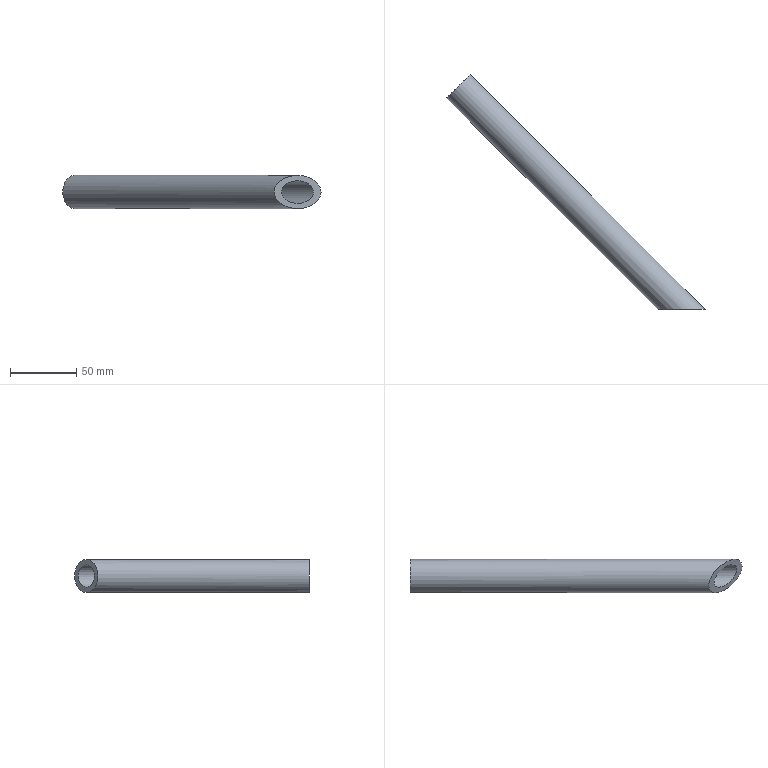Component | NX | BASE_FRAME_RND_TUBE_2 | 1 solid | 4 faces | box 194.45 x 176.78 x 25 mm | volume 62675 mm3 | plane 2 | cylinder 2 | commonest cylinder face diameters 25 x1 17 x1
STEP:
#1=CARTESIAN_POINT('',(0.,0.,0.));
#2=DIRECTION('',(0.,0.,1.));
#3=DIRECTION('',(1.,0.,0.));
#4=AXIS2_PLACEMENT_3D('',#1,#2,#3);
#5=CARTESIAN_POINT('',(-164.616,217.938,-371.5));
#6=VERTEX_POINT('',#5);
#7=CARTESIAN_POINT('',(-164.616,217.938,-380.));
#8=DIRECTION('',(0.7071,-0.7071,0.));
#9=DIRECTION('',(0.,0.,1.));
#10=AXIS2_PLACEMENT_3D('',#7,#8,#9);
#11=CIRCLE('',#10,8.5);
#12=CARTESIAN_POINT('',(-164.616,217.938,-380.));
#13=DIRECTION('',(-0.7071,0.7071,0.));
#14=DIRECTION('',(0.,0.,1.));
#15=AXIS2_PLACEMENT_3D('',#12,#13,#14);
#16=PLANE('',#15);
#17=CARTESIAN_POINT('',(8.5,0.));
#18=CARTESIAN_POINT('',(8.5,-14.722));
#19=CARTESIAN_POINT('',(-4.25,-7.361));
#20=CARTESIAN_POINT('',(-17.,-0.));
#21=CARTESIAN_POINT('',(-4.25,7.361));
#22=CARTESIAN_POINT('',(8.5,14.722));
#23=CARTESIAN_POINT('',(8.5,0.));
#24=(BOUNDED_CURVE()B_SPLINE_CURVE(2,(#17,#18,#19,#20,#21,#22,#23),.UNSPECIFIED.,.T.,.F.)B_SPLINE_CURVE_WITH_KNOTS((1,2,2,2,2,1),(-2.094,0.,2.094,4.189,6.283,8.378),.UNSPECIFIED.)CURVE()GEOMETRIC_REPRESENTATION_ITEM()RATIONAL_B_SPLINE_CURVE((1.,0.5,1.,0.5,1.,0.5,1.))REPRESENTATION_ITEM(''));
#25=(GEOMETRIC_REPRESENTATION_CONTEXT(2)PARAMETRIC_REPRESENTATION_CONTEXT()REPRESENTATION_CONTEXT('',''));
#26=DEFINITIONAL_REPRESENTATION('',(#24),#25);
#27=PCURVE('',#16,#26);
#28=CARTESIAN_POINT('',(12.161,41.161,-380.));
#29=DIRECTION('',(-0.7071,0.7071,0.));
#30=DIRECTION('',(0.,0.,1.));
#31=AXIS2_PLACEMENT_3D('',#28,#29,#30);
#32=CYLINDRICAL_SURFACE('',#31,8.5);
#33=CARTESIAN_POINT('',(6.283,250.));
#34=DIRECTION('',(-1.,0.));
#35=VECTOR('',#34,1.);
#36=LINE('',#33,#35);
#37=(GEOMETRIC_REPRESENTATION_CONTEXT(2)PARAMETRIC_REPRESENTATION_CONTEXT()REPRESENTATION_CONTEXT('',''));
#38=DEFINITIONAL_REPRESENTATION('',(#36),#37);
#39=PCURVE('',#32,#38);
#40=SURFACE_CURVE('',#11,(#27,#39),.PCURVE_S1.);
#41=EDGE_CURVE('',#6,#6,#40,.T.);
#42=ORIENTED_EDGE('',*,*,#41,.T.);
#43=EDGE_LOOP('',(#42));
#44=FACE_BOUND('',#43,.T.);
#45=CARTESIAN_POINT('',(-164.616,217.938,-367.5));
#46=VERTEX_POINT('',#45);
#47=CARTESIAN_POINT('',(-164.616,217.938,-380.));
#48=DIRECTION('',(0.7071,-0.7071,0.));
#49=DIRECTION('',(0.,0.,1.));
#50=AXIS2_PLACEMENT_3D('',#47,#48,#49);
#51=CIRCLE('',#50,12.5);
#52=CARTESIAN_POINT('',(12.5,0.));
#53=CARTESIAN_POINT('',(12.5,-21.651));
#54=CARTESIAN_POINT('',(-6.25,-10.825));
#55=CARTESIAN_POINT('',(-25.,-0.));
#56=CARTESIAN_POINT('',(-6.25,10.825));
#57=CARTESIAN_POINT('',(12.5,21.651));
#58=CARTESIAN_POINT('',(12.5,0.));
#59=(BOUNDED_CURVE()B_SPLINE_CURVE(2,(#52,#53,#54,#55,#56,#57,#58),.UNSPECIFIED.,.T.,.F.)B_SPLINE_CURVE_WITH_KNOTS((1,2,2,2,2,1),(-2.094,0.,2.094,4.189,6.283,8.378),.UNSPECIFIED.)CURVE()GEOMETRIC_REPRESENTATION_ITEM()RATIONAL_B_SPLINE_CURVE((1.,0.5,1.,0.5,1.,0.5,1.))REPRESENTATION_ITEM(''));
#60=(GEOMETRIC_REPRESENTATION_CONTEXT(2)PARAMETRIC_REPRESENTATION_CONTEXT()REPRESENTATION_CONTEXT('',''));
#61=DEFINITIONAL_REPRESENTATION('',(#59),#60);
#62=PCURVE('',#16,#61);
#63=CARTESIAN_POINT('',(12.161,41.161,-380.));
#64=DIRECTION('',(-0.7071,0.7071,0.));
#65=DIRECTION('',(0.,0.,1.));
#66=AXIS2_PLACEMENT_3D('',#63,#64,#65);
#67=CYLINDRICAL_SURFACE('',#66,12.5);
#68=CARTESIAN_POINT('',(6.283,250.));
#69=DIRECTION('',(-1.,0.));
#70=VECTOR('',#69,1.);
#71=LINE('',#68,#70);
#72=(GEOMETRIC_REPRESENTATION_CONTEXT(2)PARAMETRIC_REPRESENTATION_CONTEXT()REPRESENTATION_CONTEXT('',''));
#73=DEFINITIONAL_REPRESENTATION('',(#71),#72);
#74=PCURVE('',#67,#73);
#75=SURFACE_CURVE('',#51,(#62,#74),.PCURVE_S1.);
#76=EDGE_CURVE('',#46,#46,#75,.T.);
#77=ORIENTED_EDGE('',*,*,#76,.F.);
#78=EDGE_LOOP('',(#77));
#79=FACE_BOUND('',#78,.T.);
#80=ADVANCED_FACE('',(#44,#79),#16,.T.);
#81=CARTESIAN_POINT('',(3.322,50.,-367.5));
#82=VERTEX_POINT('',#81);
#83=CARTESIAN_POINT('',(-14.355,50.,-380.));
#84=VERTEX_POINT('',#83);
#85=CARTESIAN_POINT('',(3.322,50.,-380.));
#86=DIRECTION('',(0.,-1.,0.));
#87=DIRECTION('',(-1.,-0.,0.));
#88=AXIS2_PLACEMENT_3D('',#85,#86,#87);
#89=ELLIPSE('',#88,17.678,12.5);
#90=CARTESIAN_POINT('',(10.996,25.));
#91=CARTESIAN_POINT('',(10.9,25.006));
#92=CARTESIAN_POINT('',(10.71,24.655));
#93=CARTESIAN_POINT('',(10.424,23.16));
#94=CARTESIAN_POINT('',(10.139,20.798));
#95=CARTESIAN_POINT('',(9.853,17.764));
#96=CARTESIAN_POINT('',(9.568,14.303));
#97=CARTESIAN_POINT('',(9.282,10.697));
#98=CARTESIAN_POINT('',(8.996,7.236));
#99=CARTESIAN_POINT('',(8.711,4.202));
#100=CARTESIAN_POINT('',(8.425,1.84));
#101=CARTESIAN_POINT('',(8.14,0.3422));
#102=CARTESIAN_POINT('',(7.854,-0.1711));
#103=CARTESIAN_POINT('',(7.568,0.3422));
#104=CARTESIAN_POINT('',(7.283,1.84));
#105=CARTESIAN_POINT('',(6.997,4.202));
#106=CARTESIAN_POINT('',(6.712,7.236));
#107=CARTESIAN_POINT('',(6.426,10.697));
#108=CARTESIAN_POINT('',(6.14,14.303));
#109=CARTESIAN_POINT('',(5.855,17.764));
#110=CARTESIAN_POINT('',(5.569,20.798));
#111=CARTESIAN_POINT('',(5.284,23.16));
#112=CARTESIAN_POINT('',(4.998,24.655));
#113=CARTESIAN_POINT('',(4.808,25.006));
#114=CARTESIAN_POINT('',(4.712,25.));
#115=B_SPLINE_CURVE_WITH_KNOTS('',3,(#90,#91,#92,#93,#94,#95,#96,#97,#98,#99,#100,#101,#102,#103,#104,#105,#106,#107,#108,#109,#110,#111,#112,#113,#114),.UNSPECIFIED.,.F.,.F.,(4,1,1,1,1,1,1,1,1,1,1,1,1,1,1,1,1,1,1,1,1,1,4),(0.,0.2856,0.5712,0.8568,1.142,1.428,1.714,1.999,2.285,2.57,2.856,3.142,3.427,3.713,3.998,4.284,4.57,4.855,5.141,5.426,5.712,5.998,6.283),.QUASI_UNIFORM_KNOTS.);
#116=(GEOMETRIC_REPRESENTATION_CONTEXT(2)PARAMETRIC_REPRESENTATION_CONTEXT()REPRESENTATION_CONTEXT('',''));
#117=DEFINITIONAL_REPRESENTATION('',(#115),#116);
#118=PCURVE('',#67,#117);
#119=CARTESIAN_POINT('',(-44.865,50.,-94.));
#120=DIRECTION('',(-0.,1.,0.));
#121=DIRECTION('',(-1.,-0.,0.));
#122=AXIS2_PLACEMENT_3D('',#119,#120,#121);
#123=PLANE('',#122);
#124=CARTESIAN_POINT('',(-30.51,-286.));
#125=CARTESIAN_POINT('',(-30.51,-307.651));
#126=CARTESIAN_POINT('',(-57.026,-296.825));
#127=CARTESIAN_POINT('',(-83.543,-286.));
#128=CARTESIAN_POINT('',(-57.026,-275.175));
#129=CARTESIAN_POINT('',(-30.51,-264.349));
#130=CARTESIAN_POINT('',(-30.51,-286.));
#131=(BOUNDED_CURVE()B_SPLINE_CURVE(2,(#124,#125,#126,#127,#128,#129,#130),.UNSPECIFIED.,.T.,.F.)B_SPLINE_CURVE_WITH_KNOTS((1,2,2,2,2,1),(-2.094,0.,2.094,4.189,6.283,8.378),.UNSPECIFIED.)CURVE()GEOMETRIC_REPRESENTATION_ITEM()RATIONAL_B_SPLINE_CURVE((1.,0.5,1.,0.5,1.,0.5,1.))REPRESENTATION_ITEM(''));
#132=(GEOMETRIC_REPRESENTATION_CONTEXT(2)PARAMETRIC_REPRESENTATION_CONTEXT()REPRESENTATION_CONTEXT('',''));
#133=DEFINITIONAL_REPRESENTATION('',(#131),#132);
#134=PCURVE('',#123,#133);
#135=SURFACE_CURVE('',#89,(#118,#134),.PCURVE_S1.);
#136=EDGE_CURVE('',#82,#84,#135,.T.);
#137=ORIENTED_EDGE('',*,*,#136,.F.);
#138=CARTESIAN_POINT('',(3.322,50.,-367.5));
#139=CARTESIAN_POINT('',(-164.616,217.938,-367.5));
#140=B_SPLINE_CURVE_WITH_KNOTS('',1,(#138,#139),.UNSPECIFIED.,.F.,.F.,(2,2),(12.5,250.),.PIECEWISE_BEZIER_KNOTS.);
#141=CARTESIAN_POINT('',(6.283,0.));
#142=DIRECTION('',(0.,1.));
#143=VECTOR('',#142,1.);
#144=LINE('',#141,#143);
#145=(GEOMETRIC_REPRESENTATION_CONTEXT(2)PARAMETRIC_REPRESENTATION_CONTEXT()REPRESENTATION_CONTEXT('',''));
#146=DEFINITIONAL_REPRESENTATION('',(#144),#145);
#147=PCURVE('',#67,#146);
#148=CARTESIAN_POINT('',(0.,0.));
#149=DIRECTION('',(0.,1.));
#150=VECTOR('',#149,1.);
#151=LINE('',#148,#150);
#152=(GEOMETRIC_REPRESENTATION_CONTEXT(2)PARAMETRIC_REPRESENTATION_CONTEXT()REPRESENTATION_CONTEXT('',''));
#153=DEFINITIONAL_REPRESENTATION('',(#151),#152);
#154=PCURVE('',#67,#153);
#155=SEAM_CURVE('',#140,(#147,#154),.PCURVE_S1.);
#156=EDGE_CURVE('',#82,#46,#155,.T.);
#157=ORIENTED_EDGE('',*,*,#156,.T.);
#158=ORIENTED_EDGE('',*,*,#76,.T.);
#159=ORIENTED_EDGE('',*,*,#156,.F.);
#160=CARTESIAN_POINT('',(3.322,50.,-380.));
#161=DIRECTION('',(0.,-1.,0.));
#162=DIRECTION('',(-1.,-0.,0.));
#163=AXIS2_PLACEMENT_3D('',#160,#161,#162);
#164=ELLIPSE('',#163,17.678,12.5);
#165=CARTESIAN_POINT('',(4.712,25.));
#166=CARTESIAN_POINT('',(4.617,25.006));
#167=CARTESIAN_POINT('',(4.427,24.655));
#168=CARTESIAN_POINT('',(4.141,23.16));
#169=CARTESIAN_POINT('',(3.856,20.798));
#170=CARTESIAN_POINT('',(3.57,17.764));
#171=CARTESIAN_POINT('',(3.284,14.303));
#172=CARTESIAN_POINT('',(2.999,10.697));
#173=CARTESIAN_POINT('',(2.713,7.236));
#174=CARTESIAN_POINT('',(2.428,4.202));
#175=CARTESIAN_POINT('',(2.142,1.84));
#176=CARTESIAN_POINT('',(1.856,0.3422));
#177=CARTESIAN_POINT('',(1.571,-0.1711));
#178=CARTESIAN_POINT('',(1.285,0.3422));
#179=CARTESIAN_POINT('',(0.9996,1.84));
#180=CARTESIAN_POINT('',(0.714,4.202));
#181=CARTESIAN_POINT('',(0.4284,7.236));
#182=CARTESIAN_POINT('',(0.1428,10.697));
#183=CARTESIAN_POINT('',(-0.1428,14.303));
#184=CARTESIAN_POINT('',(-0.4284,17.764));
#185=CARTESIAN_POINT('',(-0.714,20.798));
#186=CARTESIAN_POINT('',(-0.9996,23.16));
#187=CARTESIAN_POINT('',(-1.285,24.655));
#188=CARTESIAN_POINT('',(-1.476,25.006));
#189=CARTESIAN_POINT('',(-1.571,25.));
#190=B_SPLINE_CURVE_WITH_KNOTS('',3,(#165,#166,#167,#168,#169,#170,#171,#172,#173,#174,#175,#176,#177,#178,#179,#180,#181,#182,#183,#184,#185,#186,#187,#188,#189),.UNSPECIFIED.,.F.,.F.,(4,1,1,1,1,1,1,1,1,1,1,1,1,1,1,1,1,1,1,1,1,1,4),(0.,0.2856,0.5712,0.8568,1.142,1.428,1.714,1.999,2.285,2.57,2.856,3.142,3.427,3.713,3.998,4.284,4.57,4.855,5.141,5.426,5.712,5.998,6.283),.QUASI_UNIFORM_KNOTS.);
#191=(GEOMETRIC_REPRESENTATION_CONTEXT(2)PARAMETRIC_REPRESENTATION_CONTEXT()REPRESENTATION_CONTEXT('',''));
#192=DEFINITIONAL_REPRESENTATION('',(#190),#191);
#193=PCURVE('',#67,#192);
#194=CARTESIAN_POINT('',(-30.51,-286.));
#195=CARTESIAN_POINT('',(-30.51,-307.651));
#196=CARTESIAN_POINT('',(-57.026,-296.825));
#197=CARTESIAN_POINT('',(-83.543,-286.));
#198=CARTESIAN_POINT('',(-57.026,-275.175));
#199=CARTESIAN_POINT('',(-30.51,-264.349));
#200=CARTESIAN_POINT('',(-30.51,-286.));
#201=(BOUNDED_CURVE()B_SPLINE_CURVE(2,(#194,#195,#196,#197,#198,#199,#200),.UNSPECIFIED.,.T.,.F.)B_SPLINE_CURVE_WITH_KNOTS((1,2,2,2,2,1),(-2.094,0.,2.094,4.189,6.283,8.378),.UNSPECIFIED.)CURVE()GEOMETRIC_REPRESENTATION_ITEM()RATIONAL_B_SPLINE_CURVE((1.,0.5,1.,0.5,1.,0.5,1.))REPRESENTATION_ITEM(''));
#202=(GEOMETRIC_REPRESENTATION_CONTEXT(2)PARAMETRIC_REPRESENTATION_CONTEXT()REPRESENTATION_CONTEXT('',''));
#203=DEFINITIONAL_REPRESENTATION('',(#201),#202);
#204=PCURVE('',#123,#203);
#205=SURFACE_CURVE('',#164,(#193,#204),.PCURVE_S1.);
#206=EDGE_CURVE('',#84,#82,#205,.T.);
#207=ORIENTED_EDGE('',*,*,#206,.F.);
#208=EDGE_LOOP('',(#137,#157,#158,#159,#207));
#209=FACE_BOUND('',#208,.T.);
#210=ADVANCED_FACE('',(#209),#67,.T.);
#211=CARTESIAN_POINT('',(3.322,50.,-371.5));
#212=VERTEX_POINT('',#211);
#213=CARTESIAN_POINT('',(-8.698,50.,-380.));
#214=VERTEX_POINT('',#213);
#215=CARTESIAN_POINT('',(3.322,50.,-380.));
#216=DIRECTION('',(0.,-1.,0.));
#217=DIRECTION('',(-1.,-0.,0.));
#218=AXIS2_PLACEMENT_3D('',#215,#216,#217);
#219=ELLIPSE('',#218,12.021,8.5);
#220=CARTESIAN_POINT('',(10.996,21.));
#221=CARTESIAN_POINT('',(10.9,21.004));
#222=CARTESIAN_POINT('',(10.71,20.765));
#223=CARTESIAN_POINT('',(10.424,19.749));
#224=CARTESIAN_POINT('',(10.139,18.142));
#225=CARTESIAN_POINT('',(9.853,16.079));
#226=CARTESIAN_POINT('',(9.568,13.726));
#227=CARTESIAN_POINT('',(9.282,11.274));
#228=CARTESIAN_POINT('',(8.996,8.921));
#229=CARTESIAN_POINT('',(8.711,6.857));
#230=CARTESIAN_POINT('',(8.425,5.251));
#231=CARTESIAN_POINT('',(8.14,4.233));
#232=CARTESIAN_POINT('',(7.854,3.884));
#233=CARTESIAN_POINT('',(7.568,4.233));
#234=CARTESIAN_POINT('',(7.283,5.251));
#235=CARTESIAN_POINT('',(6.997,6.857));
#236=CARTESIAN_POINT('',(6.712,8.921));
#237=CARTESIAN_POINT('',(6.426,11.274));
#238=CARTESIAN_POINT('',(6.14,13.726));
#239=CARTESIAN_POINT('',(5.855,16.079));
#240=CARTESIAN_POINT('',(5.569,18.142));
#241=CARTESIAN_POINT('',(5.284,19.749));
#242=CARTESIAN_POINT('',(4.998,20.765));
#243=CARTESIAN_POINT('',(4.808,21.004));
#244=CARTESIAN_POINT('',(4.712,21.));
#245=B_SPLINE_CURVE_WITH_KNOTS('',3,(#220,#221,#222,#223,#224,#225,#226,#227,#228,#229,#230,#231,#232,#233,#234,#235,#236,#237,#238,#239,#240,#241,#242,#243,#244),.UNSPECIFIED.,.F.,.F.,(4,1,1,1,1,1,1,1,1,1,1,1,1,1,1,1,1,1,1,1,1,1,4),(0.,0.2856,0.5712,0.8568,1.142,1.428,1.714,1.999,2.285,2.57,2.856,3.142,3.427,3.713,3.998,4.284,4.57,4.855,5.141,5.426,5.712,5.998,6.283),.QUASI_UNIFORM_KNOTS.);
#246=(GEOMETRIC_REPRESENTATION_CONTEXT(2)PARAMETRIC_REPRESENTATION_CONTEXT()REPRESENTATION_CONTEXT('',''));
#247=DEFINITIONAL_REPRESENTATION('',(#245),#246);
#248=PCURVE('',#32,#247);
#249=CARTESIAN_POINT('',(-36.166,-286.));
#250=CARTESIAN_POINT('',(-36.166,-300.722));
#251=CARTESIAN_POINT('',(-54.198,-293.361));
#252=CARTESIAN_POINT('',(-72.229,-286.));
#253=CARTESIAN_POINT('',(-54.198,-278.639));
#254=CARTESIAN_POINT('',(-36.166,-271.278));
#255=CARTESIAN_POINT('',(-36.166,-286.));
#256=(BOUNDED_CURVE()B_SPLINE_CURVE(2,(#249,#250,#251,#252,#253,#254,#255),.UNSPECIFIED.,.T.,.F.)B_SPLINE_CURVE_WITH_KNOTS((1,2,2,2,2,1),(-2.094,0.,2.094,4.189,6.283,8.378),.UNSPECIFIED.)CURVE()GEOMETRIC_REPRESENTATION_ITEM()RATIONAL_B_SPLINE_CURVE((1.,0.5,1.,0.5,1.,0.5,1.))REPRESENTATION_ITEM(''));
#257=(GEOMETRIC_REPRESENTATION_CONTEXT(2)PARAMETRIC_REPRESENTATION_CONTEXT()REPRESENTATION_CONTEXT('',''));
#258=DEFINITIONAL_REPRESENTATION('',(#256),#257);
#259=PCURVE('',#123,#258);
#260=SURFACE_CURVE('',#219,(#248,#259),.PCURVE_S1.);
#261=EDGE_CURVE('',#212,#214,#260,.T.);
#262=ORIENTED_EDGE('',*,*,#261,.F.);
#263=CARTESIAN_POINT('',(3.322,50.,-371.5));
#264=CARTESIAN_POINT('',(-164.616,217.938,-371.5));
#265=B_SPLINE_CURVE_WITH_KNOTS('',1,(#263,#264),.UNSPECIFIED.,.F.,.F.,(2,2),(12.5,250.),.PIECEWISE_BEZIER_KNOTS.);
#266=CARTESIAN_POINT('',(6.283,0.));
#267=DIRECTION('',(0.,1.));
#268=VECTOR('',#267,1.);
#269=LINE('',#266,#268);
#270=(GEOMETRIC_REPRESENTATION_CONTEXT(2)PARAMETRIC_REPRESENTATION_CONTEXT()REPRESENTATION_CONTEXT('',''));
#271=DEFINITIONAL_REPRESENTATION('',(#269),#270);
#272=PCURVE('',#32,#271);
#273=CARTESIAN_POINT('',(0.,0.));
#274=DIRECTION('',(0.,1.));
#275=VECTOR('',#274,1.);
#276=LINE('',#273,#275);
#277=(GEOMETRIC_REPRESENTATION_CONTEXT(2)PARAMETRIC_REPRESENTATION_CONTEXT()REPRESENTATION_CONTEXT('',''));
#278=DEFINITIONAL_REPRESENTATION('',(#276),#277);
#279=PCURVE('',#32,#278);
#280=SEAM_CURVE('',#265,(#272,#279),.PCURVE_S1.);
#281=EDGE_CURVE('',#212,#6,#280,.T.);
#282=ORIENTED_EDGE('',*,*,#281,.T.);
#283=ORIENTED_EDGE('',*,*,#41,.T.);
#284=ORIENTED_EDGE('',*,*,#281,.F.);
#285=CARTESIAN_POINT('',(3.322,50.,-380.));
#286=DIRECTION('',(0.,-1.,0.));
#287=DIRECTION('',(-1.,-0.,0.));
#288=AXIS2_PLACEMENT_3D('',#285,#286,#287);
#289=ELLIPSE('',#288,12.021,8.5);
#290=CARTESIAN_POINT('',(4.712,21.));
#291=CARTESIAN_POINT('',(4.617,21.004));
#292=CARTESIAN_POINT('',(4.427,20.765));
#293=CARTESIAN_POINT('',(4.141,19.749));
#294=CARTESIAN_POINT('',(3.856,18.142));
#295=CARTESIAN_POINT('',(3.57,16.079));
#296=CARTESIAN_POINT('',(3.284,13.726));
#297=CARTESIAN_POINT('',(2.999,11.274));
#298=CARTESIAN_POINT('',(2.713,8.921));
#299=CARTESIAN_POINT('',(2.428,6.857));
#300=CARTESIAN_POINT('',(2.142,5.251));
#301=CARTESIAN_POINT('',(1.856,4.233));
#302=CARTESIAN_POINT('',(1.571,3.884));
#303=CARTESIAN_POINT('',(1.285,4.233));
#304=CARTESIAN_POINT('',(0.9996,5.251));
#305=CARTESIAN_POINT('',(0.714,6.857));
#306=CARTESIAN_POINT('',(0.4284,8.921));
#307=CARTESIAN_POINT('',(0.1428,11.274));
#308=CARTESIAN_POINT('',(-0.1428,13.726));
#309=CARTESIAN_POINT('',(-0.4284,16.079));
#310=CARTESIAN_POINT('',(-0.714,18.142));
#311=CARTESIAN_POINT('',(-0.9996,19.749));
#312=CARTESIAN_POINT('',(-1.285,20.765));
#313=CARTESIAN_POINT('',(-1.476,21.004));
#314=CARTESIAN_POINT('',(-1.571,21.));
#315=B_SPLINE_CURVE_WITH_KNOTS('',3,(#290,#291,#292,#293,#294,#295,#296,#297,#298,#299,#300,#301,#302,#303,#304,#305,#306,#307,#308,#309,#310,#311,#312,#313,#314),.UNSPECIFIED.,.F.,.F.,(4,1,1,1,1,1,1,1,1,1,1,1,1,1,1,1,1,1,1,1,1,1,4),(0.,0.2856,0.5712,0.8568,1.142,1.428,1.714,1.999,2.285,2.57,2.856,3.142,3.427,3.713,3.998,4.284,4.57,4.855,5.141,5.426,5.712,5.998,6.283),.QUASI_UNIFORM_KNOTS.);
#316=(GEOMETRIC_REPRESENTATION_CONTEXT(2)PARAMETRIC_REPRESENTATION_CONTEXT()REPRESENTATION_CONTEXT('',''));
#317=DEFINITIONAL_REPRESENTATION('',(#315),#316);
#318=PCURVE('',#32,#317);
#319=CARTESIAN_POINT('',(-36.166,-286.));
#320=CARTESIAN_POINT('',(-36.166,-300.722));
#321=CARTESIAN_POINT('',(-54.198,-293.361));
#322=CARTESIAN_POINT('',(-72.229,-286.));
#323=CARTESIAN_POINT('',(-54.198,-278.639));
#324=CARTESIAN_POINT('',(-36.166,-271.278));
#325=CARTESIAN_POINT('',(-36.166,-286.));
#326=(BOUNDED_CURVE()B_SPLINE_CURVE(2,(#319,#320,#321,#322,#323,#324,#325),.UNSPECIFIED.,.T.,.F.)B_SPLINE_CURVE_WITH_KNOTS((1,2,2,2,2,1),(-2.094,0.,2.094,4.189,6.283,8.378),.UNSPECIFIED.)CURVE()GEOMETRIC_REPRESENTATION_ITEM()RATIONAL_B_SPLINE_CURVE((1.,0.5,1.,0.5,1.,0.5,1.))REPRESENTATION_ITEM(''));
#327=(GEOMETRIC_REPRESENTATION_CONTEXT(2)PARAMETRIC_REPRESENTATION_CONTEXT()REPRESENTATION_CONTEXT('',''));
#328=DEFINITIONAL_REPRESENTATION('',(#326),#327);
#329=PCURVE('',#123,#328);
#330=SURFACE_CURVE('',#289,(#318,#329),.PCURVE_S1.);
#331=EDGE_CURVE('',#214,#212,#330,.T.);
#332=ORIENTED_EDGE('',*,*,#331,.F.);
#333=EDGE_LOOP('',(#262,#282,#283,#284,#332));
#334=FACE_BOUND('',#333,.F.);
#335=ADVANCED_FACE('',(#334),#32,.F.);
#336=ORIENTED_EDGE('',*,*,#206,.T.);
#337=ORIENTED_EDGE('',*,*,#136,.T.);
#338=EDGE_LOOP('',(#336,#337));
#339=FACE_BOUND('',#338,.T.);
#340=ORIENTED_EDGE('',*,*,#331,.F.);
#341=ORIENTED_EDGE('',*,*,#261,.F.);
#342=EDGE_LOOP('',(#340,#341));
#343=FACE_BOUND('',#342,.T.);
#344=ADVANCED_FACE('',(#339,#343),#123,.F.);
#345=CLOSED_SHELL('',(#80,#210,#335,#344));
#346=MANIFOLD_SOLID_BREP('',#345);
#347=(LENGTH_UNIT()NAMED_UNIT(*)SI_UNIT(.MILLI.,.METRE.));
#348=UNCERTAINTY_MEASURE_WITH_UNIT(LENGTH_MEASURE(0.001),#347,'','');
#349=(NAMED_UNIT(*)PLANE_ANGLE_UNIT()SI_UNIT($,.RADIAN.));
#350=(NAMED_UNIT(*)SI_UNIT($,.STERADIAN.)SOLID_ANGLE_UNIT());
#351=(GEOMETRIC_REPRESENTATION_CONTEXT(3)GLOBAL_UNCERTAINTY_ASSIGNED_CONTEXT((#348))GLOBAL_UNIT_ASSIGNED_CONTEXT((#347,#349,#350))REPRESENTATION_CONTEXT('',''));
#352=ADVANCED_BREP_SHAPE_REPRESENTATION('',(#4,#346),#351);